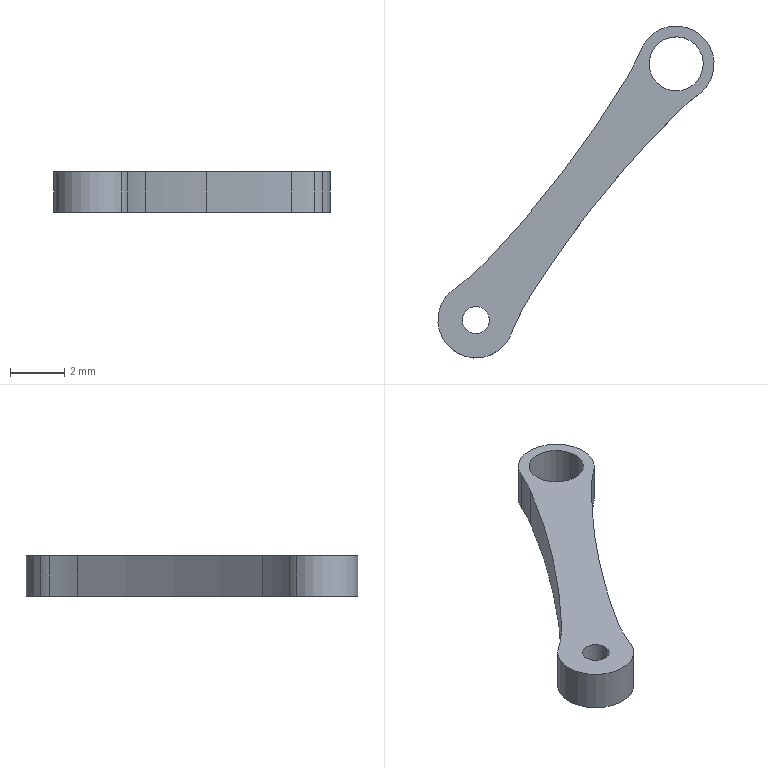Component | SolidWorks | ConnectingRod-3 | 1 solid | 19 faces | box 10.19 x 12.25 x 1.5 mm | volume 40 mm3 | cylinder 17 | plane 2 | commonest cylinder face diameters 2.8 x6 16 x4 76 x3 2 x2 1 x2
build123d program:
from build123d import *
from build123d.topology import SkipClean

# Parameters (mm, degrees)
BOSS_EXTRUDE1_DEPTH = 0.25
BOSS_EXTRUDE2_DEPTH = 0.75
SKETCH4_R           = 1
SKETCH4_R_2         = 0.5
CUT_EXTRUDE1_DEPTH  = 2.5
SKETCH5_R           = 0.5
SKETCH5_R_2         = 1
BOSS_EXTRUDE3_DEPTH = 1.5
SKETCH6_OUTSIDE_W   = 19.828
SKETCH6_OUTSIDE_H   = 7.828
CUT_EXTRUDE2_DEPTH  = 10


with BuildPart() as part:
    # Sketch1 → Boss-Extrude1 (new, symmetric)
    with BuildSketch(Plane(origin=(0, 0, 0), x_dir=(1, 0, 0), z_dir=(0, 1, 0))):
        with BuildLine():
            Line((0, 1.4), (12, 1.4))
            ThreePointArc((12, 1.4), (13.4, 0), (12, -1.4))
            Line((12, -1.4), (0, -1.4))
            ThreePointArc((0, -1.4), (-1.4, 0), (0, 1.4))
        make_face()
    extrude(amount=BOSS_EXTRUDE1_DEPTH, both=True)

    # Sketch3 → Boss-Extrude2 (add, symmetric)
    with BuildSketch(Plane(origin=(0, 0, 0), x_dir=(1, 0, 0), z_dir=(0, 1, 0))):
        with BuildLine():
            Line((1.326, 0.45), (10.674, 0.45))
            ThreePointArc((10.674, 0.45), (13.4, 0), (10.674, -0.45))
            Line((10.674, -0.45), (1.326, -0.45))
            ThreePointArc((1.326, -0.45), (-1.4, 0), (1.326, 0.45))
        make_face()
    extrude(amount=BOSS_EXTRUDE2_DEPTH, both=True)

    # Sketch4 → Cut-Extrude1 (cut)
    with BuildSketch(Plane(origin=(0, 0.75, 0), x_dir=(1, 0, 0), z_dir=(0, 1, 0))):
        with Locations(Location((0, 0, 0), (0, 0, 270))):
            Circle(SKETCH4_R)
        with Locations(Location((12, 0, 0), (0, 0, 270))):
            Circle(SKETCH4_R_2)
    extrude(amount=-CUT_EXTRUDE1_DEPTH, mode=Mode.SUBTRACT)

    # Sketch5 → Boss-Extrude3 (add)
    # profile 1 of 3: a face of its own
    with BuildSketch(Plane(origin=(0, 0.75, 0), x_dir=(1, 0, 0), z_dir=(0, 1, 0))):
        with BuildLine():
            Line((1.326, -0.45), (10.674, -0.45))
            ThreePointArc((10.674, -0.45), (13.4, 0), (10.674, 0.45))
            Line((10.674, 0.45), (1.326, 0.45))
            ThreePointArc((1.326, 0.45), (-1.4, 0), (1.326, -0.45))
        make_face()
        with Locations(Location((12, 0, 0), (0, 0, 270))):
            Circle(SKETCH5_R, mode=Mode.SUBTRACT)
        with Locations(Location((0, 0, 0), (0, 0, 270))):
            Circle(SKETCH5_R_2, mode=Mode.SUBTRACT)
    # profile 2 of 3: a face of its own
    with BuildSketch(Plane(origin=(0, 0.75, 0), x_dir=(1, 0, 0), z_dir=(0, 1, 0))):
        with BuildLine():
            Line((0, -1.4), (12, -1.4))
            ThreePointArc((12, -1.4), (11.185, -1.138), (10.674, -0.45))
            Line((10.674, -0.45), (1.326, -0.45))
            ThreePointArc((1.326, -0.45), (0.8155, -1.138), (0, -1.4))
        make_face()
    # profile 3 of 3: a face of its own
    with BuildSketch(Plane(origin=(0, 0.75, 0), x_dir=(1, 0, 0), z_dir=(0, 1, 0))):
        with BuildLine():
            Line((1.326, 0.45), (10.674, 0.45))
            ThreePointArc((10.674, 0.45), (11.185, 1.138), (12, 1.4))
            Line((12, 1.4), (0, 1.4))
            ThreePointArc((0, 1.4), (0.8155, 1.138), (1.326, 0.45))
        make_face()
    extrude(amount=-BOSS_EXTRUDE3_DEPTH)

    # Sketch6 outside → Cut-Extrude2 (cut)
    with SkipClean():  # the faces are left unmerged after this step: merging them gives an invalid solid
        with BuildSketch(Plane.XZ.offset(0.75)):
            with Locations((6, 0)):
                Rectangle(SKETCH6_OUTSIDE_W, SKETCH6_OUTSIDE_H)
            with BuildLine():
                ThreePointArc((0.3708, 1.35), (0.9343, 1.217), (1.506, 1.125))
                ThreePointArc((1.506, 1.125), (5.802, 0.8385), (10.104, 1.04))
                ThreePointArc((10.104, 1.04), (10.856, 1.154), (11.594, 1.34))
                ThreePointArc((11.594, 1.34), (13.4, 0), (11.594, -1.34))
                ThreePointArc((11.594, -1.34), (10.856, -1.154), (10.104, -1.04))
                ThreePointArc((10.104, -1.04), (5.802, -0.8385), (1.506, -1.125))
                ThreePointArc((1.506, -1.125), (0.9343, -1.217), (0.3708, -1.35))
                ThreePointArc((0.3708, -1.35), (-1.4, 0), (0.3708, 1.35))
            make_face(mode=Mode.SUBTRACT)
        extrude(amount=-CUT_EXTRUDE2_DEPTH, mode=Mode.SUBTRACT)


solid = part.part

# Placed as in the assembly
solid = solid.moved(Location((-1.962, 7.074, 35.5), (-90, -51.974, 180)))
STEP:
#1=COLOUR_RGB('',0.7922,0.8196,0.9333);
#2=FILL_AREA_STYLE_COLOUR('',#1);
#3=FILL_AREA_STYLE('',(#2));
#4=SURFACE_STYLE_FILL_AREA(#3);
#5=SURFACE_SIDE_STYLE('',(#4));
#6=SURFACE_STYLE_USAGE(.BOTH.,#5);
#7=PRESENTATION_STYLE_ASSIGNMENT((#6));
#8=CARTESIAN_POINT('',(-0.2012,0.0666,1.368));
#9=VERTEX_POINT('',#8);
#10=CARTESIAN_POINT('',(-0.29,-0.06005,1.368));
#11=VERTEX_POINT('',#10);
#12=CARTESIAN_POINT('',(0.9773,-0.855,1.368));
#13=DIRECTION('',(-0.,0.,1.));
#14=DIRECTION('',(0.7877,-0.616,0.));
#15=AXIS2_PLACEMENT_3D('',#12,#13,#14);
#16=CIRCLE('',#15,1.496);
#17=EDGE_CURVE('',#9,#11,#16,.T.);
#18=ORIENTED_EDGE('',*,*,#17,.F.);
#19=CARTESIAN_POINT('',(-0.2012,0.0666,1.427));
#20=VERTEX_POINT('',#19);
#21=CARTESIAN_POINT('',(-0.2012,0.0666,1.033));
#22=DIRECTION('',(-0.,0.,1.));
#23=VECTOR('',#22,39.37);
#24=LINE('',#21,#23);
#25=EDGE_CURVE('',#9,#20,#24,.T.);
#26=ORIENTED_EDGE('',*,*,#25,.T.);
#27=CARTESIAN_POINT('',(-0.29,-0.06005,1.427));
#28=VERTEX_POINT('',#27);
#29=CARTESIAN_POINT('',(0.9773,-0.855,1.427));
#30=DIRECTION('',(0.,-0.,-1.));
#31=DIRECTION('',(-0.7877,0.616,0.));
#32=AXIS2_PLACEMENT_3D('',#29,#30,#31);
#33=CIRCLE('',#32,1.496);
#34=EDGE_CURVE('',#28,#20,#33,.T.);
#35=ORIENTED_EDGE('',*,*,#34,.F.);
#36=CARTESIAN_POINT('',(-0.29,-0.06005,1.033));
#37=DIRECTION('',(-0.,0.,1.));
#38=VECTOR('',#37,39.37);
#39=LINE('',#36,#38);
#40=EDGE_CURVE('',#11,#28,#39,.T.);
#41=ORIENTED_EDGE('',*,*,#40,.F.);
#42=EDGE_LOOP('',(#18,#26,#35,#41));
#43=FACE_OUTER_BOUND('',#42,.T.);
#44=CARTESIAN_POINT('',(0.9773,-0.855,1.033));
#45=DIRECTION('',(-0.,0.,1.));
#46=DIRECTION('',(-0.7877,0.616,0.));
#47=AXIS2_PLACEMENT_3D('',#44,#45,#46);
#48=CYLINDRICAL_SURFACE('',#47,1.496);
#49=ADVANCED_FACE('',(#43),#48,.F.);
#50=CARTESIAN_POINT('',(-0.1083,0.3028,1.427));
#51=VERTEX_POINT('',#50);
#52=CARTESIAN_POINT('',(-0.04624,0.2543,1.427));
#53=VERTEX_POINT('',#52);
#54=CARTESIAN_POINT('',(-0.07725,0.2785,1.427));
#55=DIRECTION('',(0.,-0.,-1.));
#56=DIRECTION('',(0.7877,-0.616,0.));
#57=AXIS2_PLACEMENT_3D('',#54,#55,#56);
#58=CIRCLE('',#57,0.03937);
#59=EDGE_CURVE('',#51,#53,#58,.T.);
#60=ORIENTED_EDGE('',*,*,#59,.F.);
#61=CARTESIAN_POINT('',(-0.1083,0.3028,1.368));
#62=VERTEX_POINT('',#61);
#63=CARTESIAN_POINT('',(-0.1083,0.3028,1.467));
#64=DIRECTION('',(0.,-0.,-1.));
#65=VECTOR('',#64,39.37);
#66=LINE('',#63,#65);
#67=EDGE_CURVE('',#51,#62,#66,.T.);
#68=ORIENTED_EDGE('',*,*,#67,.T.);
#69=CARTESIAN_POINT('',(-0.04624,0.2543,1.368));
#70=VERTEX_POINT('',#69);
#71=CARTESIAN_POINT('',(-0.07725,0.2785,1.368));
#72=DIRECTION('',(0.,-0.,-1.));
#73=DIRECTION('',(0.7877,-0.616,0.));
#74=AXIS2_PLACEMENT_3D('',#71,#72,#73);
#75=CIRCLE('',#74,0.03937);
#76=EDGE_CURVE('',#62,#70,#75,.T.);
#77=ORIENTED_EDGE('',*,*,#76,.T.);
#78=CARTESIAN_POINT('',(-0.04624,0.2543,1.467));
#79=DIRECTION('',(0.,-0.,-1.));
#80=VECTOR('',#79,39.37);
#81=LINE('',#78,#80);
#82=EDGE_CURVE('',#53,#70,#81,.T.);
#83=ORIENTED_EDGE('',*,*,#82,.F.);
#84=EDGE_LOOP('',(#60,#68,#77,#83));
#85=FACE_OUTER_BOUND('',#84,.T.);
#86=CARTESIAN_POINT('',(-0.07725,0.2785,1.467));
#87=DIRECTION('',(0.,-0.,-1.));
#88=DIRECTION('',(0.7877,-0.616,0.));
#89=AXIS2_PLACEMENT_3D('',#86,#87,#88);
#90=CYLINDRICAL_SURFACE('',#89,0.03937);
#91=ADVANCED_FACE('',(#85),#90,.F.);
#92=CARTESIAN_POINT('',(-0.3838,-0.08152,1.427));
#93=VERTEX_POINT('',#92);
#94=CARTESIAN_POINT('',(-0.3528,-0.1058,1.427));
#95=VERTEX_POINT('',#94);
#96=CARTESIAN_POINT('',(-0.3683,-0.09364,1.427));
#97=DIRECTION('',(0.,-0.,-1.));
#98=DIRECTION('',(0.7877,-0.616,0.));
#99=AXIS2_PLACEMENT_3D('',#96,#97,#98);
#100=CIRCLE('',#99,0.01969);
#101=EDGE_CURVE('',#93,#95,#100,.T.);
#102=ORIENTED_EDGE('',*,*,#101,.F.);
#103=CARTESIAN_POINT('',(-0.3838,-0.08152,1.368));
#104=VERTEX_POINT('',#103);
#105=CARTESIAN_POINT('',(-0.3838,-0.08152,1.467));
#106=DIRECTION('',(0.,-0.,-1.));
#107=VECTOR('',#106,39.37);
#108=LINE('',#105,#107);
#109=EDGE_CURVE('',#93,#104,#108,.T.);
#110=ORIENTED_EDGE('',*,*,#109,.T.);
#111=CARTESIAN_POINT('',(-0.3528,-0.1058,1.368));
#112=VERTEX_POINT('',#111);
#113=CARTESIAN_POINT('',(-0.3683,-0.09364,1.368));
#114=DIRECTION('',(0.,-0.,-1.));
#115=DIRECTION('',(0.7877,-0.616,0.));
#116=AXIS2_PLACEMENT_3D('',#113,#114,#115);
#117=CIRCLE('',#116,0.01969);
#118=EDGE_CURVE('',#104,#112,#117,.T.);
#119=ORIENTED_EDGE('',*,*,#118,.T.);
#120=CARTESIAN_POINT('',(-0.3528,-0.1058,1.467));
#121=DIRECTION('',(0.,-0.,-1.));
#122=VECTOR('',#121,39.37);
#123=LINE('',#120,#122);
#124=EDGE_CURVE('',#95,#112,#123,.T.);
#125=ORIENTED_EDGE('',*,*,#124,.F.);
#126=EDGE_LOOP('',(#102,#110,#119,#125));
#127=FACE_OUTER_BOUND('',#126,.T.);
#128=CARTESIAN_POINT('',(-0.3683,-0.09364,1.467));
#129=DIRECTION('',(0.,-0.,-1.));
#130=DIRECTION('',(0.7877,-0.616,0.));
#131=AXIS2_PLACEMENT_3D('',#128,#129,#130);
#132=CYLINDRICAL_SURFACE('',#131,0.01969);
#133=ADVANCED_FACE('',(#127),#132,.F.);
#134=CARTESIAN_POINT('',(-0.3249,-0.1276,1.368));
#135=VERTEX_POINT('',#134);
#136=CARTESIAN_POINT('',(-0.4117,-0.05969,1.368));
#137=VERTEX_POINT('',#136);
#138=CARTESIAN_POINT('',(-0.3683,-0.09364,1.368));
#139=DIRECTION('',(0.,-0.,-1.));
#140=DIRECTION('',(0.7877,-0.616,0.));
#141=AXIS2_PLACEMENT_3D('',#138,#139,#140);
#142=CIRCLE('',#141,0.05512);
#143=EDGE_CURVE('',#135,#137,#142,.T.);
#144=ORIENTED_EDGE('',*,*,#143,.F.);
#145=CARTESIAN_POINT('',(-0.3249,-0.1276,1.427));
#146=VERTEX_POINT('',#145);
#147=CARTESIAN_POINT('',(-0.3249,-0.1276,1.388));
#148=DIRECTION('',(-0.,0.,1.));
#149=VECTOR('',#148,39.37);
#150=LINE('',#147,#149);
#151=EDGE_CURVE('',#135,#146,#150,.T.);
#152=ORIENTED_EDGE('',*,*,#151,.T.);
#153=CARTESIAN_POINT('',(-0.4117,-0.05969,1.427));
#154=VERTEX_POINT('',#153);
#155=CARTESIAN_POINT('',(-0.3683,-0.09364,1.427));
#156=DIRECTION('',(0.,-0.,-1.));
#157=DIRECTION('',(0.7877,-0.616,0.));
#158=AXIS2_PLACEMENT_3D('',#155,#156,#157);
#159=CIRCLE('',#158,0.05512);
#160=EDGE_CURVE('',#146,#154,#159,.T.);
#161=ORIENTED_EDGE('',*,*,#160,.T.);
#162=CARTESIAN_POINT('',(-0.4117,-0.05969,1.388));
#163=DIRECTION('',(-0.,0.,1.));
#164=VECTOR('',#163,39.37);
#165=LINE('',#162,#164);
#166=EDGE_CURVE('',#137,#154,#165,.T.);
#167=ORIENTED_EDGE('',*,*,#166,.F.);
#168=EDGE_LOOP('',(#144,#152,#161,#167));
#169=FACE_OUTER_BOUND('',#168,.T.);
#170=CARTESIAN_POINT('',(-0.3683,-0.09364,1.388));
#171=DIRECTION('',(-0.,0.,1.));
#172=DIRECTION('',(-0.7877,0.616,0.));
#173=AXIS2_PLACEMENT_3D('',#170,#171,#172);
#174=CYLINDRICAL_SURFACE('',#173,0.05512);
#175=ADVANCED_FACE('',(#169),#174,.T.);
#176=CARTESIAN_POINT('',(-0.4,-0.04857,1.368));
#177=VERTEX_POINT('',#176);
#178=CARTESIAN_POINT('',(-0.3683,-0.09364,1.368));
#179=DIRECTION('',(0.,-0.,-1.));
#180=DIRECTION('',(0.7877,-0.616,0.));
#181=AXIS2_PLACEMENT_3D('',#178,#179,#180);
#182=CIRCLE('',#181,0.05512);
#183=EDGE_CURVE('',#137,#177,#182,.T.);
#184=ORIENTED_EDGE('',*,*,#183,.F.);
#185=ORIENTED_EDGE('',*,*,#166,.T.);
#186=CARTESIAN_POINT('',(-0.4,-0.04857,1.427));
#187=VERTEX_POINT('',#186);
#188=CARTESIAN_POINT('',(-0.3683,-0.09364,1.427));
#189=DIRECTION('',(0.,-0.,-1.));
#190=DIRECTION('',(0.7877,-0.616,0.));
#191=AXIS2_PLACEMENT_3D('',#188,#189,#190);
#192=CIRCLE('',#191,0.05512);
#193=EDGE_CURVE('',#154,#187,#192,.T.);
#194=ORIENTED_EDGE('',*,*,#193,.T.);
#195=CARTESIAN_POINT('',(-0.4,-0.04857,1.033));
#196=DIRECTION('',(-0.,0.,1.));
#197=VECTOR('',#196,39.37);
#198=LINE('',#195,#197);
#199=EDGE_CURVE('',#177,#187,#198,.T.);
#200=ORIENTED_EDGE('',*,*,#199,.F.);
#201=EDGE_LOOP('',(#184,#185,#194,#200));
#202=FACE_OUTER_BOUND('',#201,.T.);
#203=CARTESIAN_POINT('',(-0.3683,-0.09364,1.388));
#204=DIRECTION('',(-0.,0.,1.));
#205=DIRECTION('',(-0.7877,0.616,0.));
#206=AXIS2_PLACEMENT_3D('',#203,#204,#205);
#207=CYLINDRICAL_SURFACE('',#206,0.05512);
#208=ADVANCED_FACE('',(#202),#207,.T.);
#209=CARTESIAN_POINT('',(-0.03383,0.2446,1.368));
#210=VERTEX_POINT('',#209);
#211=CARTESIAN_POINT('',(-0.04438,0.2343,1.368));
#212=VERTEX_POINT('',#211);
#213=CARTESIAN_POINT('',(-0.07725,0.2785,1.368));
#214=DIRECTION('',(0.,-0.,-1.));
#215=DIRECTION('',(0.7877,-0.616,0.));
#216=AXIS2_PLACEMENT_3D('',#213,#214,#215);
#217=CIRCLE('',#216,0.05512);
#218=EDGE_CURVE('',#210,#212,#217,.T.);
#219=ORIENTED_EDGE('',*,*,#218,.F.);
#220=CARTESIAN_POINT('',(-0.03383,0.2446,1.427));
#221=VERTEX_POINT('',#220);
#222=CARTESIAN_POINT('',(-0.03383,0.2446,1.388));
#223=DIRECTION('',(-0.,0.,1.));
#224=VECTOR('',#223,39.37);
#225=LINE('',#222,#224);
#226=EDGE_CURVE('',#210,#221,#225,.T.);
#227=ORIENTED_EDGE('',*,*,#226,.T.);
#228=CARTESIAN_POINT('',(-0.04438,0.2343,1.427));
#229=VERTEX_POINT('',#228);
#230=CARTESIAN_POINT('',(-0.07725,0.2785,1.427));
#231=DIRECTION('',(0.,-0.,-1.));
#232=DIRECTION('',(0.7877,-0.616,0.));
#233=AXIS2_PLACEMENT_3D('',#230,#231,#232);
#234=CIRCLE('',#233,0.05512);
#235=EDGE_CURVE('',#221,#229,#234,.T.);
#236=ORIENTED_EDGE('',*,*,#235,.T.);
#237=CARTESIAN_POINT('',(-0.04438,0.2343,1.033));
#238=DIRECTION('',(-0.,0.,1.));
#239=VECTOR('',#238,39.37);
#240=LINE('',#237,#239);
#241=EDGE_CURVE('',#212,#229,#240,.T.);
#242=ORIENTED_EDGE('',*,*,#241,.F.);
#243=EDGE_LOOP('',(#219,#227,#236,#242));
#244=FACE_OUTER_BOUND('',#243,.T.);
#245=CARTESIAN_POINT('',(-0.07725,0.2785,1.388));
#246=DIRECTION('',(-0.,0.,1.));
#247=DIRECTION('',(-0.7877,0.616,0.));
#248=AXIS2_PLACEMENT_3D('',#245,#246,#247);
#249=CYLINDRICAL_SURFACE('',#248,0.05512);
#250=ADVANCED_FACE('',(#244),#249,.T.);
#251=ORIENTED_EDGE('',*,*,#226,.F.);
#252=CARTESIAN_POINT('',(-0.1207,0.3125,1.368));
#253=VERTEX_POINT('',#252);
#254=CARTESIAN_POINT('',(-0.07725,0.2785,1.368));
#255=DIRECTION('',(0.,-0.,-1.));
#256=DIRECTION('',(0.7877,-0.616,0.));
#257=AXIS2_PLACEMENT_3D('',#254,#255,#256);
#258=CIRCLE('',#257,0.05512);
#259=EDGE_CURVE('',#253,#210,#258,.T.);
#260=ORIENTED_EDGE('',*,*,#259,.F.);
#261=CARTESIAN_POINT('',(-0.1207,0.3125,1.427));
#262=VERTEX_POINT('',#261);
#263=CARTESIAN_POINT('',(-0.1207,0.3125,1.388));
#264=DIRECTION('',(-0.,0.,1.));
#265=VECTOR('',#264,39.37);
#266=LINE('',#263,#265);
#267=EDGE_CURVE('',#253,#262,#266,.T.);
#268=ORIENTED_EDGE('',*,*,#267,.T.);
#269=CARTESIAN_POINT('',(-0.07725,0.2785,1.427));
#270=DIRECTION('',(0.,-0.,-1.));
#271=DIRECTION('',(0.7877,-0.616,0.));
#272=AXIS2_PLACEMENT_3D('',#269,#270,#271);
#273=CIRCLE('',#272,0.05512);
#274=EDGE_CURVE('',#262,#221,#273,.T.);
#275=ORIENTED_EDGE('',*,*,#274,.T.);
#276=EDGE_LOOP('',(#251,#260,#268,#275));
#277=FACE_OUTER_BOUND('',#276,.T.);
#278=CARTESIAN_POINT('',(-0.07725,0.2785,1.388));
#279=DIRECTION('',(-0.,0.,1.));
#280=DIRECTION('',(-0.7877,0.616,0.));
#281=AXIS2_PLACEMENT_3D('',#278,#279,#280);
#282=CYLINDRICAL_SURFACE('',#281,0.05512);
#283=ADVANCED_FACE('',(#277),#282,.T.);
#284=ORIENTED_EDGE('',*,*,#267,.F.);
#285=CARTESIAN_POINT('',(-0.1281,0.2998,1.368));
#286=VERTEX_POINT('',#285);
#287=CARTESIAN_POINT('',(-0.07725,0.2785,1.368));
#288=DIRECTION('',(0.,-0.,-1.));
#289=DIRECTION('',(0.7877,-0.616,0.));
#290=AXIS2_PLACEMENT_3D('',#287,#288,#289);
#291=CIRCLE('',#290,0.05512);
#292=EDGE_CURVE('',#286,#253,#291,.T.);
#293=ORIENTED_EDGE('',*,*,#292,.F.);
#294=CARTESIAN_POINT('',(-0.1281,0.2998,1.427));
#295=VERTEX_POINT('',#294);
#296=CARTESIAN_POINT('',(-0.1281,0.2998,1.033));
#297=DIRECTION('',(-0.,0.,1.));
#298=VECTOR('',#297,39.37);
#299=LINE('',#296,#298);
#300=EDGE_CURVE('',#286,#295,#299,.T.);
#301=ORIENTED_EDGE('',*,*,#300,.T.);
#302=CARTESIAN_POINT('',(-0.07725,0.2785,1.427));
#303=DIRECTION('',(0.,-0.,-1.));
#304=DIRECTION('',(0.7877,-0.616,0.));
#305=AXIS2_PLACEMENT_3D('',#302,#303,#304);
#306=CIRCLE('',#305,0.05512);
#307=EDGE_CURVE('',#295,#262,#306,.T.);
#308=ORIENTED_EDGE('',*,*,#307,.T.);
#309=EDGE_LOOP('',(#284,#293,#301,#308));
#310=FACE_OUTER_BOUND('',#309,.T.);
#311=CARTESIAN_POINT('',(-0.07725,0.2785,1.388));
#312=DIRECTION('',(-0.,0.,1.));
#313=DIRECTION('',(-0.7877,0.616,0.));
#314=AXIS2_PLACEMENT_3D('',#311,#312,#313);
#315=CYLINDRICAL_SURFACE('',#314,0.05512);
#316=ADVANCED_FACE('',(#310),#315,.T.);
#317=ORIENTED_EDGE('',*,*,#151,.F.);
#318=CARTESIAN_POINT('',(-0.3169,-0.1136,1.368));
#319=VERTEX_POINT('',#318);
#320=CARTESIAN_POINT('',(-0.3683,-0.09364,1.368));
#321=DIRECTION('',(0.,-0.,-1.));
#322=DIRECTION('',(0.7877,-0.616,0.));
#323=AXIS2_PLACEMENT_3D('',#320,#321,#322);
#324=CIRCLE('',#323,0.05512);
#325=EDGE_CURVE('',#319,#135,#324,.T.);
#326=ORIENTED_EDGE('',*,*,#325,.F.);
#327=CARTESIAN_POINT('',(-0.3169,-0.1136,1.427));
#328=VERTEX_POINT('',#327);
#329=CARTESIAN_POINT('',(-0.3169,-0.1136,1.033));
#330=DIRECTION('',(-0.,0.,1.));
#331=VECTOR('',#330,39.37);
#332=LINE('',#329,#331);
#333=EDGE_CURVE('',#319,#328,#332,.T.);
#334=ORIENTED_EDGE('',*,*,#333,.T.);
#335=CARTESIAN_POINT('',(-0.3683,-0.09364,1.427));
#336=DIRECTION('',(0.,-0.,-1.));
#337=DIRECTION('',(0.7877,-0.616,0.));
#338=AXIS2_PLACEMENT_3D('',#335,#336,#337);
#339=CIRCLE('',#338,0.05512);
#340=EDGE_CURVE('',#328,#146,#339,.T.);
#341=ORIENTED_EDGE('',*,*,#340,.T.);
#342=EDGE_LOOP('',(#317,#326,#334,#341));
#343=FACE_OUTER_BOUND('',#342,.T.);
#344=CARTESIAN_POINT('',(-0.3683,-0.09364,1.388));
#345=DIRECTION('',(-0.,0.,1.));
#346=DIRECTION('',(-0.7877,0.616,0.));
#347=AXIS2_PLACEMENT_3D('',#344,#345,#346);
#348=CYLINDRICAL_SURFACE('',#347,0.05512);
#349=ADVANCED_FACE('',(#343),#348,.T.);
#350=CARTESIAN_POINT('',(-0.3545,-0.009613,1.427));
#351=VERTEX_POINT('',#350);
#352=CARTESIAN_POINT('',(-0.5813,0.209,1.427));
#353=DIRECTION('',(0.,-0.,-1.));
#354=DIRECTION('',(0.7877,-0.616,0.));
#355=AXIS2_PLACEMENT_3D('',#352,#353,#354);
#356=CIRCLE('',#355,0.315);
#357=EDGE_CURVE('',#351,#187,#356,.T.);
#358=ORIENTED_EDGE('',*,*,#357,.T.);
#359=ORIENTED_EDGE('',*,*,#193,.F.);
#360=ORIENTED_EDGE('',*,*,#160,.F.);
#361=ORIENTED_EDGE('',*,*,#340,.F.);
#362=CARTESIAN_POINT('',(-0.02323,-0.2274,1.427));
#363=DIRECTION('',(0.,-0.,-1.));
#364=DIRECTION('',(-0.7877,0.616,0.));
#365=AXIS2_PLACEMENT_3D('',#362,#363,#364);
#366=CIRCLE('',#365,0.315);
#367=EDGE_CURVE('',#328,#28,#366,.T.);
#368=ORIENTED_EDGE('',*,*,#367,.T.);
#369=ORIENTED_EDGE('',*,*,#34,.T.);
#370=CARTESIAN_POINT('',(-0.07889,0.2045,1.427));
#371=VERTEX_POINT('',#370);
#372=CARTESIAN_POINT('',(0.9773,-0.855,1.427));
#373=DIRECTION('',(0.,-0.,-1.));
#374=DIRECTION('',(-0.7877,0.616,0.));
#375=AXIS2_PLACEMENT_3D('',#372,#373,#374);
#376=CIRCLE('',#375,1.496);
#377=EDGE_CURVE('',#20,#371,#376,.T.);
#378=ORIENTED_EDGE('',*,*,#377,.T.);
#379=CARTESIAN_POINT('',(0.1435,-0.01854,1.427));
#380=DIRECTION('',(0.,-0.,-1.));
#381=DIRECTION('',(-0.7877,0.616,0.));
#382=AXIS2_PLACEMENT_3D('',#379,#380,#381);
#383=CIRCLE('',#382,0.315);
#384=EDGE_CURVE('',#371,#229,#383,.T.);
#385=ORIENTED_EDGE('',*,*,#384,.T.);
#386=ORIENTED_EDGE('',*,*,#235,.F.);
#387=ORIENTED_EDGE('',*,*,#274,.F.);
#388=ORIENTED_EDGE('',*,*,#307,.F.);
#389=CARTESIAN_POINT('',(-0.1487,0.2591,1.427));
#390=VERTEX_POINT('',#389);
#391=CARTESIAN_POINT('',(-0.4187,0.4211,1.427));
#392=DIRECTION('',(0.,-0.,-1.));
#393=DIRECTION('',(0.7877,-0.616,0.));
#394=AXIS2_PLACEMENT_3D('',#391,#392,#393);
#395=CIRCLE('',#394,0.315);
#396=EDGE_CURVE('',#295,#390,#395,.T.);
#397=ORIENTED_EDGE('',*,*,#396,.T.);
#398=CARTESIAN_POINT('',(-1.432,1.029,1.427));
#399=DIRECTION('',(0.,-0.,-1.));
#400=DIRECTION('',(0.7877,-0.616,0.));
#401=AXIS2_PLACEMENT_3D('',#398,#399,#400);
#402=CIRCLE('',#401,1.496);
#403=EDGE_CURVE('',#390,#351,#402,.T.);
#404=ORIENTED_EDGE('',*,*,#403,.T.);
#405=EDGE_LOOP('',(#358,#359,#360,#361,#368,#369,#378,#385,#386,#387,#388,#397,#404));
#406=FACE_OUTER_BOUND('',#405,.T.);
#407=CARTESIAN_POINT('',(-0.07725,0.2785,1.427));
#408=DIRECTION('',(0.,-0.,-1.));
#409=DIRECTION('',(0.7877,-0.616,0.));
#410=AXIS2_PLACEMENT_3D('',#407,#408,#409);
#411=CIRCLE('',#410,0.03937);
#412=EDGE_CURVE('',#53,#51,#411,.T.);
#413=ORIENTED_EDGE('',*,*,#412,.T.);
#414=ORIENTED_EDGE('',*,*,#59,.T.);
#415=EDGE_LOOP('',(#413,#414));
#416=FACE_BOUND('',#415,.T.);
#417=CARTESIAN_POINT('',(-0.3683,-0.09364,1.427));
#418=DIRECTION('',(0.,-0.,-1.));
#419=DIRECTION('',(0.7877,-0.616,0.));
#420=AXIS2_PLACEMENT_3D('',#417,#418,#419);
#421=CIRCLE('',#420,0.01969);
#422=EDGE_CURVE('',#95,#93,#421,.T.);
#423=ORIENTED_EDGE('',*,*,#422,.T.);
#424=ORIENTED_EDGE('',*,*,#101,.T.);
#425=EDGE_LOOP('',(#423,#424));
#426=FACE_BOUND('',#425,.T.);
#427=CARTESIAN_POINT('',(-0.3683,-0.09364,1.427));
#428=DIRECTION('',(0.,-0.,-1.));
#429=DIRECTION('',(0.7877,-0.616,0.));
#430=AXIS2_PLACEMENT_3D('',#427,#428,#429);
#431=PLANE('',#430);
#432=ADVANCED_FACE('',(#406,#416,#426),#431,.F.);
#433=ORIENTED_EDGE('',*,*,#325,.T.);
#434=ORIENTED_EDGE('',*,*,#143,.T.);
#435=ORIENTED_EDGE('',*,*,#183,.T.);
#436=CARTESIAN_POINT('',(-0.3545,-0.009613,1.368));
#437=VERTEX_POINT('',#436);
#438=CARTESIAN_POINT('',(-0.5813,0.209,1.368));
#439=DIRECTION('',(-0.,0.,1.));
#440=DIRECTION('',(0.7877,-0.616,0.));
#441=AXIS2_PLACEMENT_3D('',#438,#439,#440);
#442=CIRCLE('',#441,0.315);
#443=EDGE_CURVE('',#177,#437,#442,.T.);
#444=ORIENTED_EDGE('',*,*,#443,.T.);
#445=CARTESIAN_POINT('',(-0.1487,0.2591,1.368));
#446=VERTEX_POINT('',#445);
#447=CARTESIAN_POINT('',(-1.432,1.029,1.368));
#448=DIRECTION('',(-0.,0.,1.));
#449=DIRECTION('',(0.7877,-0.616,0.));
#450=AXIS2_PLACEMENT_3D('',#447,#448,#449);
#451=CIRCLE('',#450,1.496);
#452=EDGE_CURVE('',#437,#446,#451,.T.);
#453=ORIENTED_EDGE('',*,*,#452,.T.);
#454=CARTESIAN_POINT('',(-0.4187,0.4211,1.368));
#455=DIRECTION('',(-0.,0.,1.));
#456=DIRECTION('',(0.7877,-0.616,0.));
#457=AXIS2_PLACEMENT_3D('',#454,#455,#456);
#458=CIRCLE('',#457,0.315);
#459=EDGE_CURVE('',#446,#286,#458,.T.);
#460=ORIENTED_EDGE('',*,*,#459,.T.);
#461=ORIENTED_EDGE('',*,*,#292,.T.);
#462=ORIENTED_EDGE('',*,*,#259,.T.);
#463=ORIENTED_EDGE('',*,*,#218,.T.);
#464=CARTESIAN_POINT('',(-0.07889,0.2045,1.368));
#465=VERTEX_POINT('',#464);
#466=CARTESIAN_POINT('',(0.1435,-0.01854,1.368));
#467=DIRECTION('',(-0.,0.,1.));
#468=DIRECTION('',(0.7877,-0.616,0.));
#469=AXIS2_PLACEMENT_3D('',#466,#467,#468);
#470=CIRCLE('',#469,0.315);
#471=EDGE_CURVE('',#212,#465,#470,.T.);
#472=ORIENTED_EDGE('',*,*,#471,.T.);
#473=CARTESIAN_POINT('',(0.9773,-0.855,1.368));
#474=DIRECTION('',(-0.,0.,1.));
#475=DIRECTION('',(0.7877,-0.616,0.));
#476=AXIS2_PLACEMENT_3D('',#473,#474,#475);
#477=CIRCLE('',#476,1.496);
#478=EDGE_CURVE('',#465,#9,#477,.T.);
#479=ORIENTED_EDGE('',*,*,#478,.T.);
#480=ORIENTED_EDGE('',*,*,#17,.T.);
#481=CARTESIAN_POINT('',(-0.02323,-0.2274,1.368));
#482=DIRECTION('',(-0.,0.,1.));
#483=DIRECTION('',(0.7877,-0.616,0.));
#484=AXIS2_PLACEMENT_3D('',#481,#482,#483);
#485=CIRCLE('',#484,0.315);
#486=EDGE_CURVE('',#11,#319,#485,.T.);
#487=ORIENTED_EDGE('',*,*,#486,.T.);
#488=EDGE_LOOP('',(#433,#434,#435,#444,#453,#460,#461,#462,#463,#472,#479,#480,#487));
#489=FACE_OUTER_BOUND('',#488,.T.);
#490=CARTESIAN_POINT('',(-0.07725,0.2785,1.368));
#491=DIRECTION('',(0.,-0.,-1.));
#492=DIRECTION('',(0.7877,-0.616,0.));
#493=AXIS2_PLACEMENT_3D('',#490,#491,#492);
#494=CIRCLE('',#493,0.03937);
#495=EDGE_CURVE('',#70,#62,#494,.T.);
#496=ORIENTED_EDGE('',*,*,#495,.F.);
#497=ORIENTED_EDGE('',*,*,#76,.F.);
#498=EDGE_LOOP('',(#496,#497));
#499=FACE_BOUND('',#498,.T.);
#500=CARTESIAN_POINT('',(-0.3683,-0.09364,1.368));
#501=DIRECTION('',(0.,-0.,-1.));
#502=DIRECTION('',(0.7877,-0.616,0.));
#503=AXIS2_PLACEMENT_3D('',#500,#501,#502);
#504=CIRCLE('',#503,0.01969);
#505=EDGE_CURVE('',#112,#104,#504,.T.);
#506=ORIENTED_EDGE('',*,*,#505,.F.);
#507=ORIENTED_EDGE('',*,*,#118,.F.);
#508=EDGE_LOOP('',(#506,#507));
#509=FACE_BOUND('',#508,.T.);
#510=CARTESIAN_POINT('',(-0.3683,-0.09364,1.368));
#511=DIRECTION('',(0.,-0.,-1.));
#512=DIRECTION('',(0.7877,-0.616,0.));
#513=AXIS2_PLACEMENT_3D('',#510,#511,#512);
#514=PLANE('',#513);
#515=ADVANCED_FACE('',(#489,#499,#509),#514,.T.);
#516=ORIENTED_EDGE('',*,*,#109,.F.);
#517=ORIENTED_EDGE('',*,*,#422,.F.);
#518=ORIENTED_EDGE('',*,*,#124,.T.);
#519=ORIENTED_EDGE('',*,*,#505,.T.);
#520=EDGE_LOOP('',(#516,#517,#518,#519));
#521=FACE_OUTER_BOUND('',#520,.T.);
#522=CARTESIAN_POINT('',(-0.3683,-0.09364,1.467));
#523=DIRECTION('',(0.,-0.,-1.));
#524=DIRECTION('',(0.7877,-0.616,0.));
#525=AXIS2_PLACEMENT_3D('',#522,#523,#524);
#526=CYLINDRICAL_SURFACE('',#525,0.01969);
#527=ADVANCED_FACE('',(#521),#526,.F.);
#528=ORIENTED_EDGE('',*,*,#67,.F.);
#529=ORIENTED_EDGE('',*,*,#412,.F.);
#530=ORIENTED_EDGE('',*,*,#82,.T.);
#531=ORIENTED_EDGE('',*,*,#495,.T.);
#532=EDGE_LOOP('',(#528,#529,#530,#531));
#533=FACE_OUTER_BOUND('',#532,.T.);
#534=CARTESIAN_POINT('',(-0.07725,0.2785,1.467));
#535=DIRECTION('',(0.,-0.,-1.));
#536=DIRECTION('',(0.7877,-0.616,0.));
#537=AXIS2_PLACEMENT_3D('',#534,#535,#536);
#538=CYLINDRICAL_SURFACE('',#537,0.03937);
#539=ADVANCED_FACE('',(#533),#538,.F.);
#540=ORIENTED_EDGE('',*,*,#40,.T.);
#541=ORIENTED_EDGE('',*,*,#367,.F.);
#542=ORIENTED_EDGE('',*,*,#333,.F.);
#543=ORIENTED_EDGE('',*,*,#486,.F.);
#544=EDGE_LOOP('',(#540,#541,#542,#543));
#545=FACE_OUTER_BOUND('',#544,.T.);
#546=CARTESIAN_POINT('',(-0.02323,-0.2274,1.033));
#547=DIRECTION('',(-0.,0.,1.));
#548=DIRECTION('',(-0.7877,0.616,0.));
#549=AXIS2_PLACEMENT_3D('',#546,#547,#548);
#550=CYLINDRICAL_SURFACE('',#549,0.315);
#551=ADVANCED_FACE('',(#545),#550,.F.);
#552=ORIENTED_EDGE('',*,*,#241,.T.);
#553=ORIENTED_EDGE('',*,*,#384,.F.);
#554=CARTESIAN_POINT('',(-0.07889,0.2045,1.033));
#555=DIRECTION('',(-0.,0.,1.));
#556=VECTOR('',#555,39.37);
#557=LINE('',#554,#556);
#558=EDGE_CURVE('',#465,#371,#557,.T.);
#559=ORIENTED_EDGE('',*,*,#558,.F.);
#560=ORIENTED_EDGE('',*,*,#471,.F.);
#561=EDGE_LOOP('',(#552,#553,#559,#560));
#562=FACE_OUTER_BOUND('',#561,.T.);
#563=CARTESIAN_POINT('',(0.1435,-0.01854,1.033));
#564=DIRECTION('',(-0.,0.,1.));
#565=DIRECTION('',(-0.7877,0.616,0.));
#566=AXIS2_PLACEMENT_3D('',#563,#564,#565);
#567=CYLINDRICAL_SURFACE('',#566,0.315);
#568=ADVANCED_FACE('',(#562),#567,.F.);
#569=ORIENTED_EDGE('',*,*,#25,.F.);
#570=ORIENTED_EDGE('',*,*,#478,.F.);
#571=ORIENTED_EDGE('',*,*,#558,.T.);
#572=ORIENTED_EDGE('',*,*,#377,.F.);
#573=EDGE_LOOP('',(#569,#570,#571,#572));
#574=FACE_OUTER_BOUND('',#573,.T.);
#575=CARTESIAN_POINT('',(0.9773,-0.855,1.033));
#576=DIRECTION('',(-0.,0.,1.));
#577=DIRECTION('',(-0.7877,0.616,0.));
#578=AXIS2_PLACEMENT_3D('',#575,#576,#577);
#579=CYLINDRICAL_SURFACE('',#578,1.496);
#580=ADVANCED_FACE('',(#574),#579,.F.);
#581=ORIENTED_EDGE('',*,*,#199,.T.);
#582=ORIENTED_EDGE('',*,*,#357,.F.);
#583=CARTESIAN_POINT('',(-0.3545,-0.009613,1.033));
#584=DIRECTION('',(-0.,0.,1.));
#585=VECTOR('',#584,39.37);
#586=LINE('',#583,#585);
#587=EDGE_CURVE('',#437,#351,#586,.T.);
#588=ORIENTED_EDGE('',*,*,#587,.F.);
#589=ORIENTED_EDGE('',*,*,#443,.F.);
#590=EDGE_LOOP('',(#581,#582,#588,#589));
#591=FACE_OUTER_BOUND('',#590,.T.);
#592=CARTESIAN_POINT('',(-0.5813,0.209,1.033));
#593=DIRECTION('',(-0.,0.,1.));
#594=DIRECTION('',(-0.7877,0.616,0.));
#595=AXIS2_PLACEMENT_3D('',#592,#593,#594);
#596=CYLINDRICAL_SURFACE('',#595,0.315);
#597=ADVANCED_FACE('',(#591),#596,.F.);
#598=ORIENTED_EDGE('',*,*,#587,.T.);
#599=ORIENTED_EDGE('',*,*,#403,.F.);
#600=CARTESIAN_POINT('',(-0.1487,0.2591,1.033));
#601=DIRECTION('',(-0.,0.,1.));
#602=VECTOR('',#601,39.37);
#603=LINE('',#600,#602);
#604=EDGE_CURVE('',#446,#390,#603,.T.);
#605=ORIENTED_EDGE('',*,*,#604,.F.);
#606=ORIENTED_EDGE('',*,*,#452,.F.);
#607=EDGE_LOOP('',(#598,#599,#605,#606));
#608=FACE_OUTER_BOUND('',#607,.T.);
#609=CARTESIAN_POINT('',(-1.432,1.029,1.033));
#610=DIRECTION('',(-0.,0.,1.));
#611=DIRECTION('',(-0.7877,0.616,0.));
#612=AXIS2_PLACEMENT_3D('',#609,#610,#611);
#613=CYLINDRICAL_SURFACE('',#612,1.496);
#614=ADVANCED_FACE('',(#608),#613,.F.);
#615=ORIENTED_EDGE('',*,*,#604,.T.);
#616=ORIENTED_EDGE('',*,*,#396,.F.);
#617=ORIENTED_EDGE('',*,*,#300,.F.);
#618=ORIENTED_EDGE('',*,*,#459,.F.);
#619=EDGE_LOOP('',(#615,#616,#617,#618));
#620=FACE_OUTER_BOUND('',#619,.T.);
#621=CARTESIAN_POINT('',(-0.4187,0.4211,1.033));
#622=DIRECTION('',(-0.,0.,1.));
#623=DIRECTION('',(-0.7877,0.616,0.));
#624=AXIS2_PLACEMENT_3D('',#621,#622,#623);
#625=CYLINDRICAL_SURFACE('',#624,0.315);
#626=ADVANCED_FACE('',(#620),#625,.F.);
#627=CLOSED_SHELL('',(#49,#91,#133,#175,#208,#250,#283,#316,#349,#432,#515,#527,#539,#551,#568,#580,#597,#614,#626));
#628=MANIFOLD_SOLID_BREP('',#627);
#629=STYLED_ITEM('',(#7),#628);
#630=(LENGTH_UNIT()NAMED_UNIT(*)SI_UNIT($,.METRE.));
#631=LENGTH_MEASURE_WITH_UNIT(LENGTH_MEASURE(0.0254),#630);
#632=DIMENSIONAL_EXPONENTS(1.,0.,0.,0.,0.,0.,0.);
#633=(CONVERSION_BASED_UNIT('',#631)LENGTH_UNIT()NAMED_UNIT(#632));
#634=UNCERTAINTY_MEASURE_WITH_UNIT(LENGTH_MEASURE(0.00001),#633,'','');
#635=(NAMED_UNIT(*)PLANE_ANGLE_UNIT()SI_UNIT($,.RADIAN.));
#636=(NAMED_UNIT(*)SI_UNIT($,.STERADIAN.)SOLID_ANGLE_UNIT());
#637=(GEOMETRIC_REPRESENTATION_CONTEXT(3)GLOBAL_UNCERTAINTY_ASSIGNED_CONTEXT((#634))GLOBAL_UNIT_ASSIGNED_CONTEXT((#633,#635,#636))REPRESENTATION_CONTEXT('',''));
#638=MECHANICAL_DESIGN_GEOMETRIC_PRESENTATION_REPRESENTATION('',(#629),#637);
#639=PRESENTATION_LAYER_ASSIGNMENT('','',(#629));
#640=CARTESIAN_POINT('',(0.,0.,0.));
#641=DIRECTION('',(0.,0.,1.));
#642=DIRECTION('',(1.,0.,0.));
#643=AXIS2_PLACEMENT_3D('',#640,#641,#642);
#644=(LENGTH_UNIT()NAMED_UNIT(*)SI_UNIT($,.METRE.));
#645=LENGTH_MEASURE_WITH_UNIT(LENGTH_MEASURE(0.0254),#644);
#646=DIMENSIONAL_EXPONENTS(1.,0.,0.,0.,0.,0.,0.);
#647=(CONVERSION_BASED_UNIT('',#645)LENGTH_UNIT()NAMED_UNIT(#646));
#648=UNCERTAINTY_MEASURE_WITH_UNIT(LENGTH_MEASURE(0.00001),#647,'','');
#649=(NAMED_UNIT(*)PLANE_ANGLE_UNIT()SI_UNIT($,.RADIAN.));
#650=(NAMED_UNIT(*)SI_UNIT($,.STERADIAN.)SOLID_ANGLE_UNIT());
#651=(GEOMETRIC_REPRESENTATION_CONTEXT(3)GLOBAL_UNCERTAINTY_ASSIGNED_CONTEXT((#648))GLOBAL_UNIT_ASSIGNED_CONTEXT((#647,#649,#650))REPRESENTATION_CONTEXT('',''));
#652=ADVANCED_BREP_SHAPE_REPRESENTATION('',(#628,#643),#651);